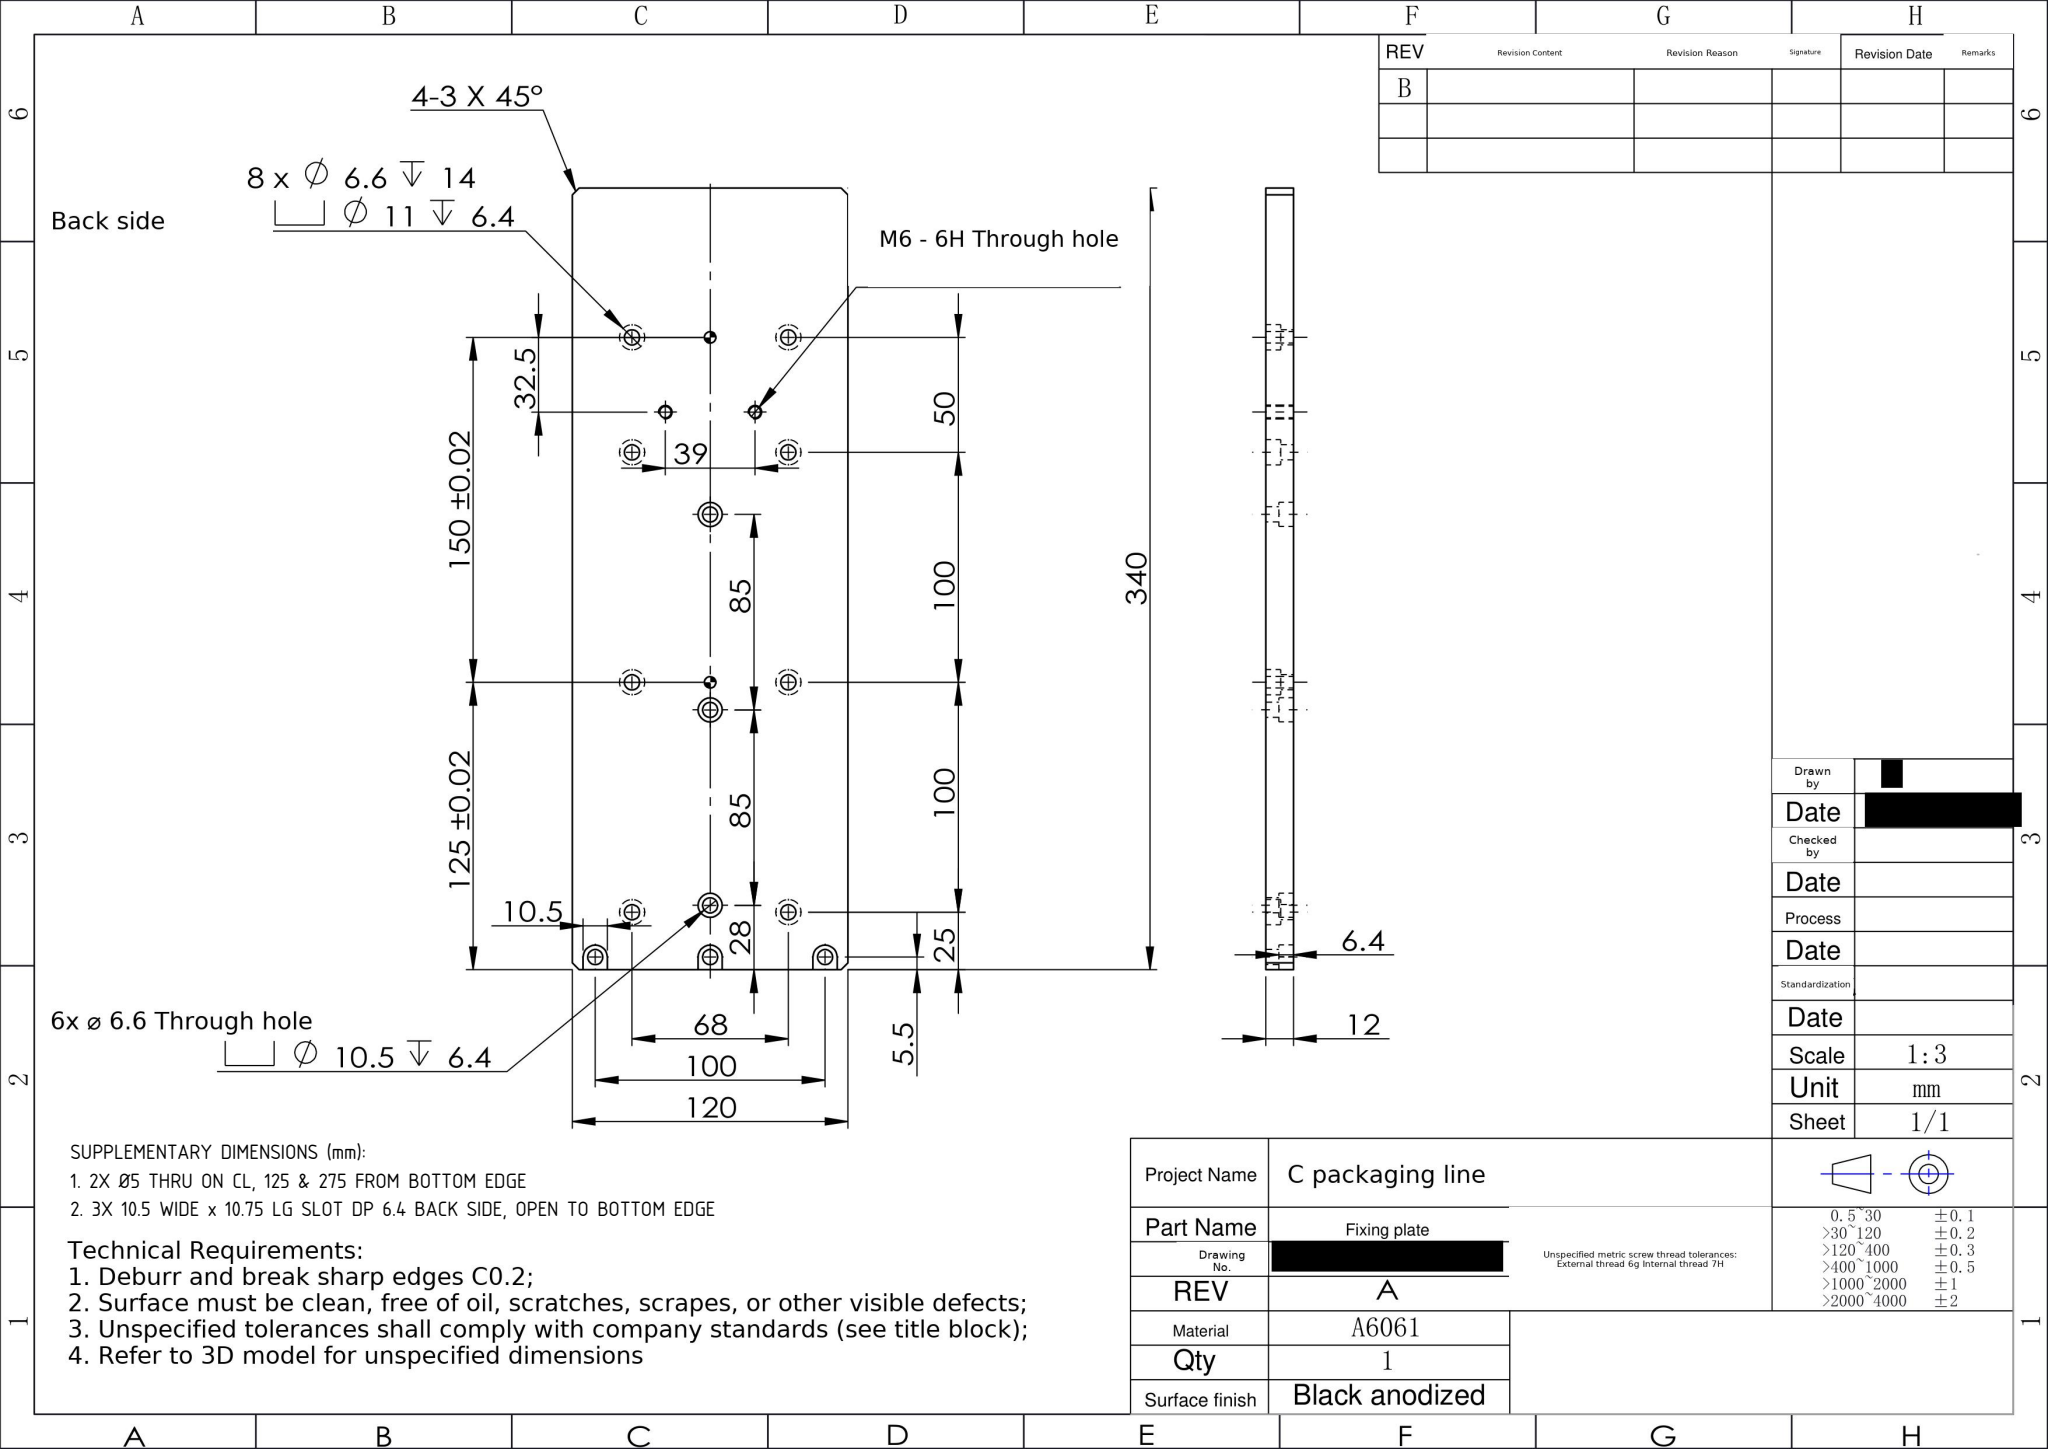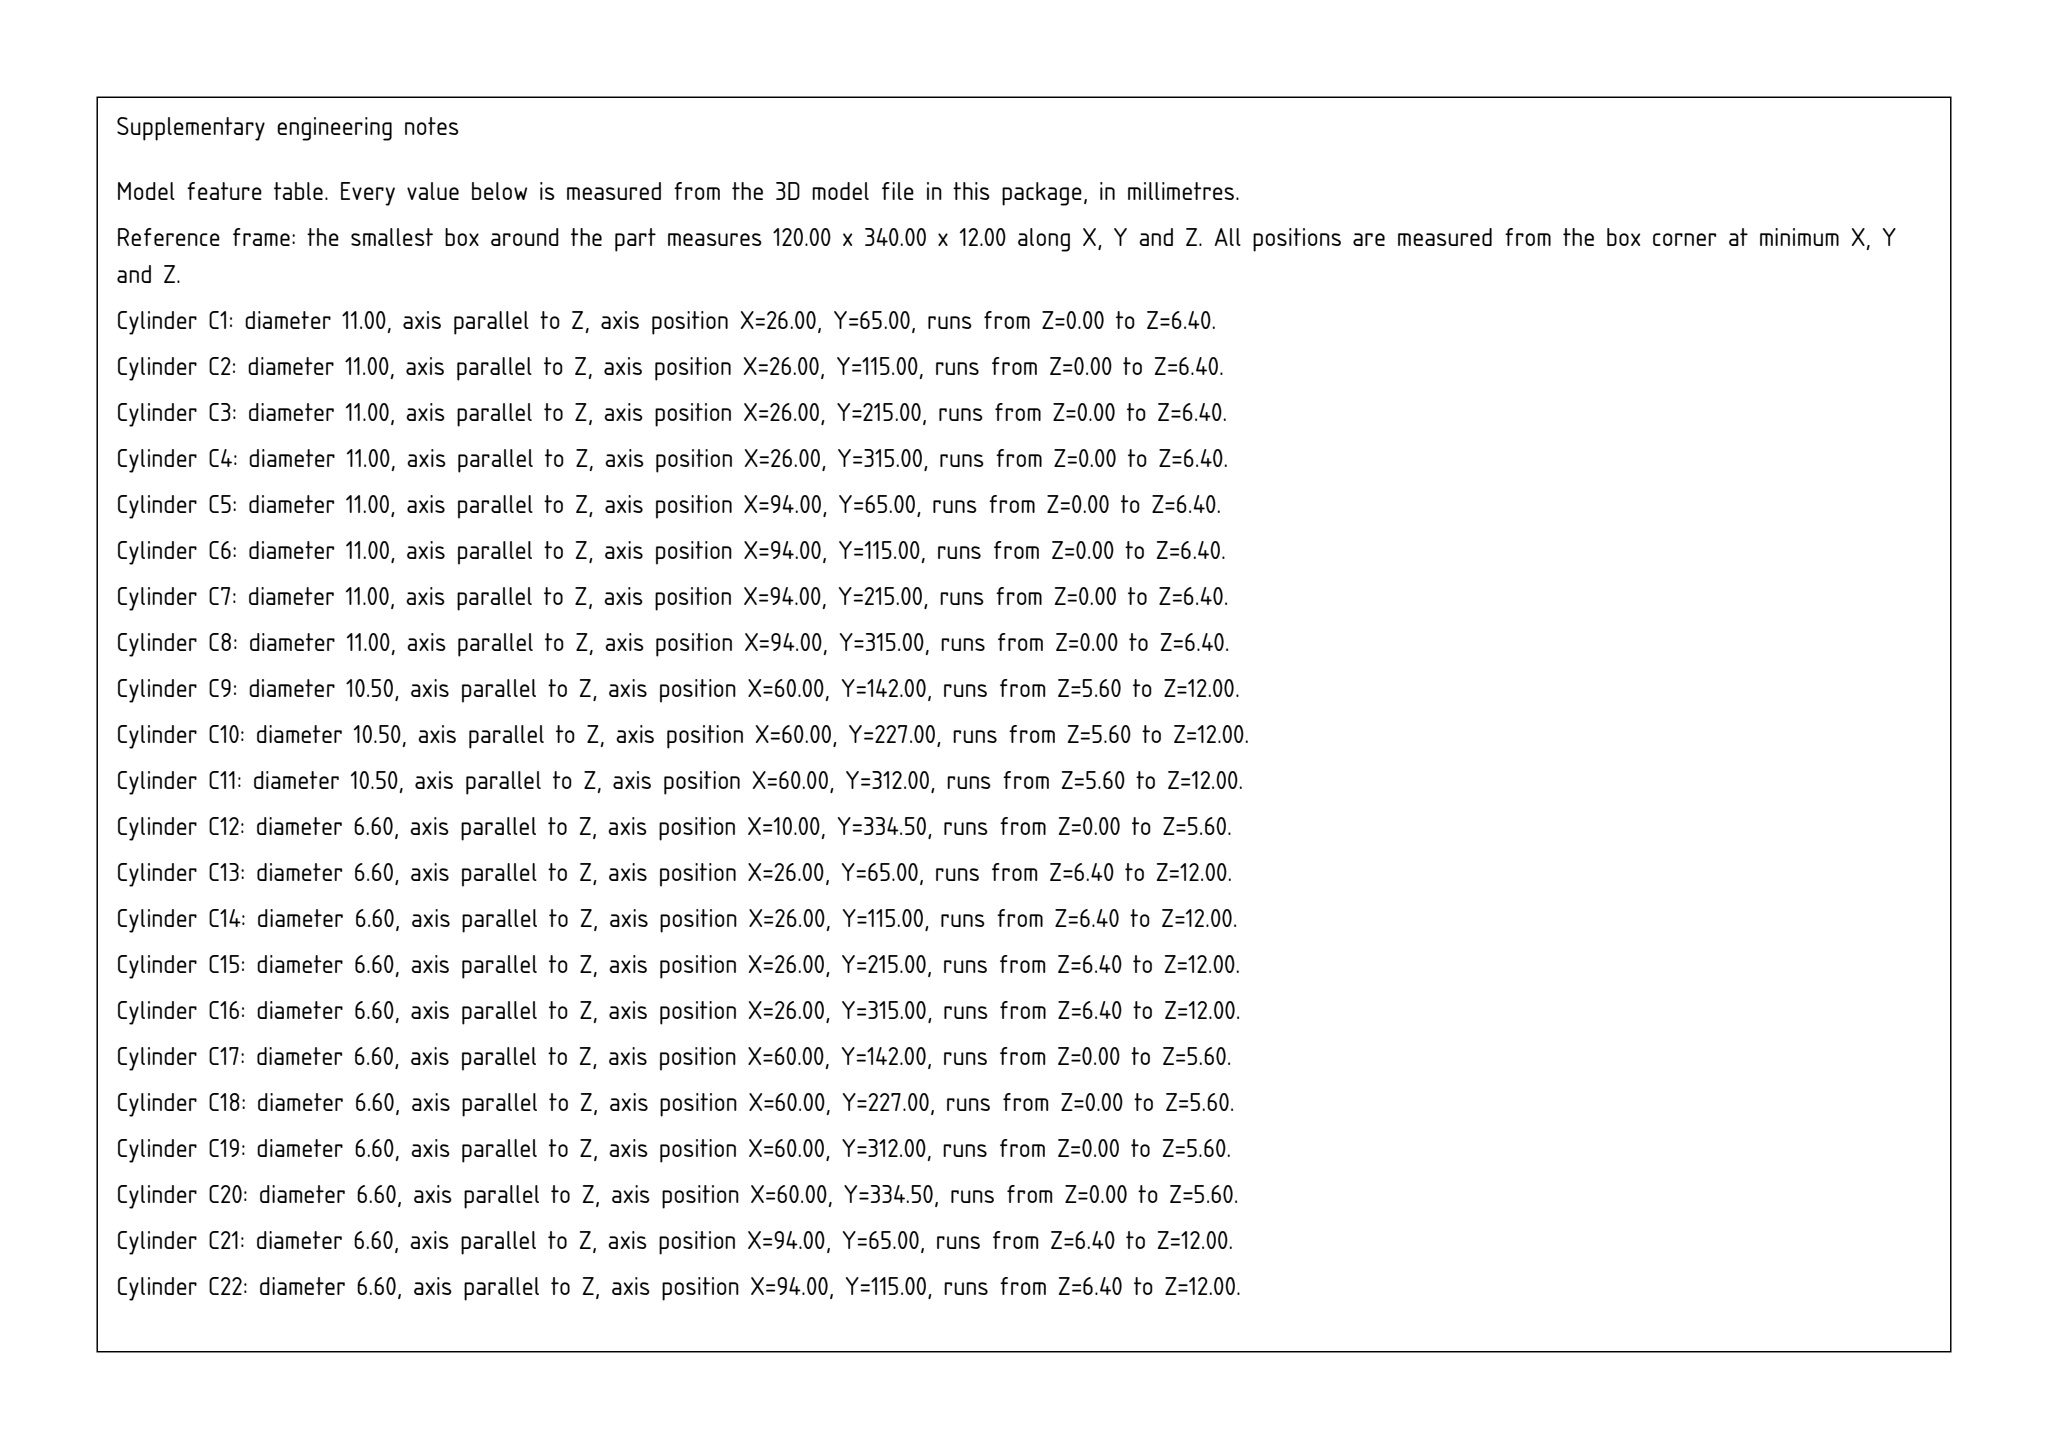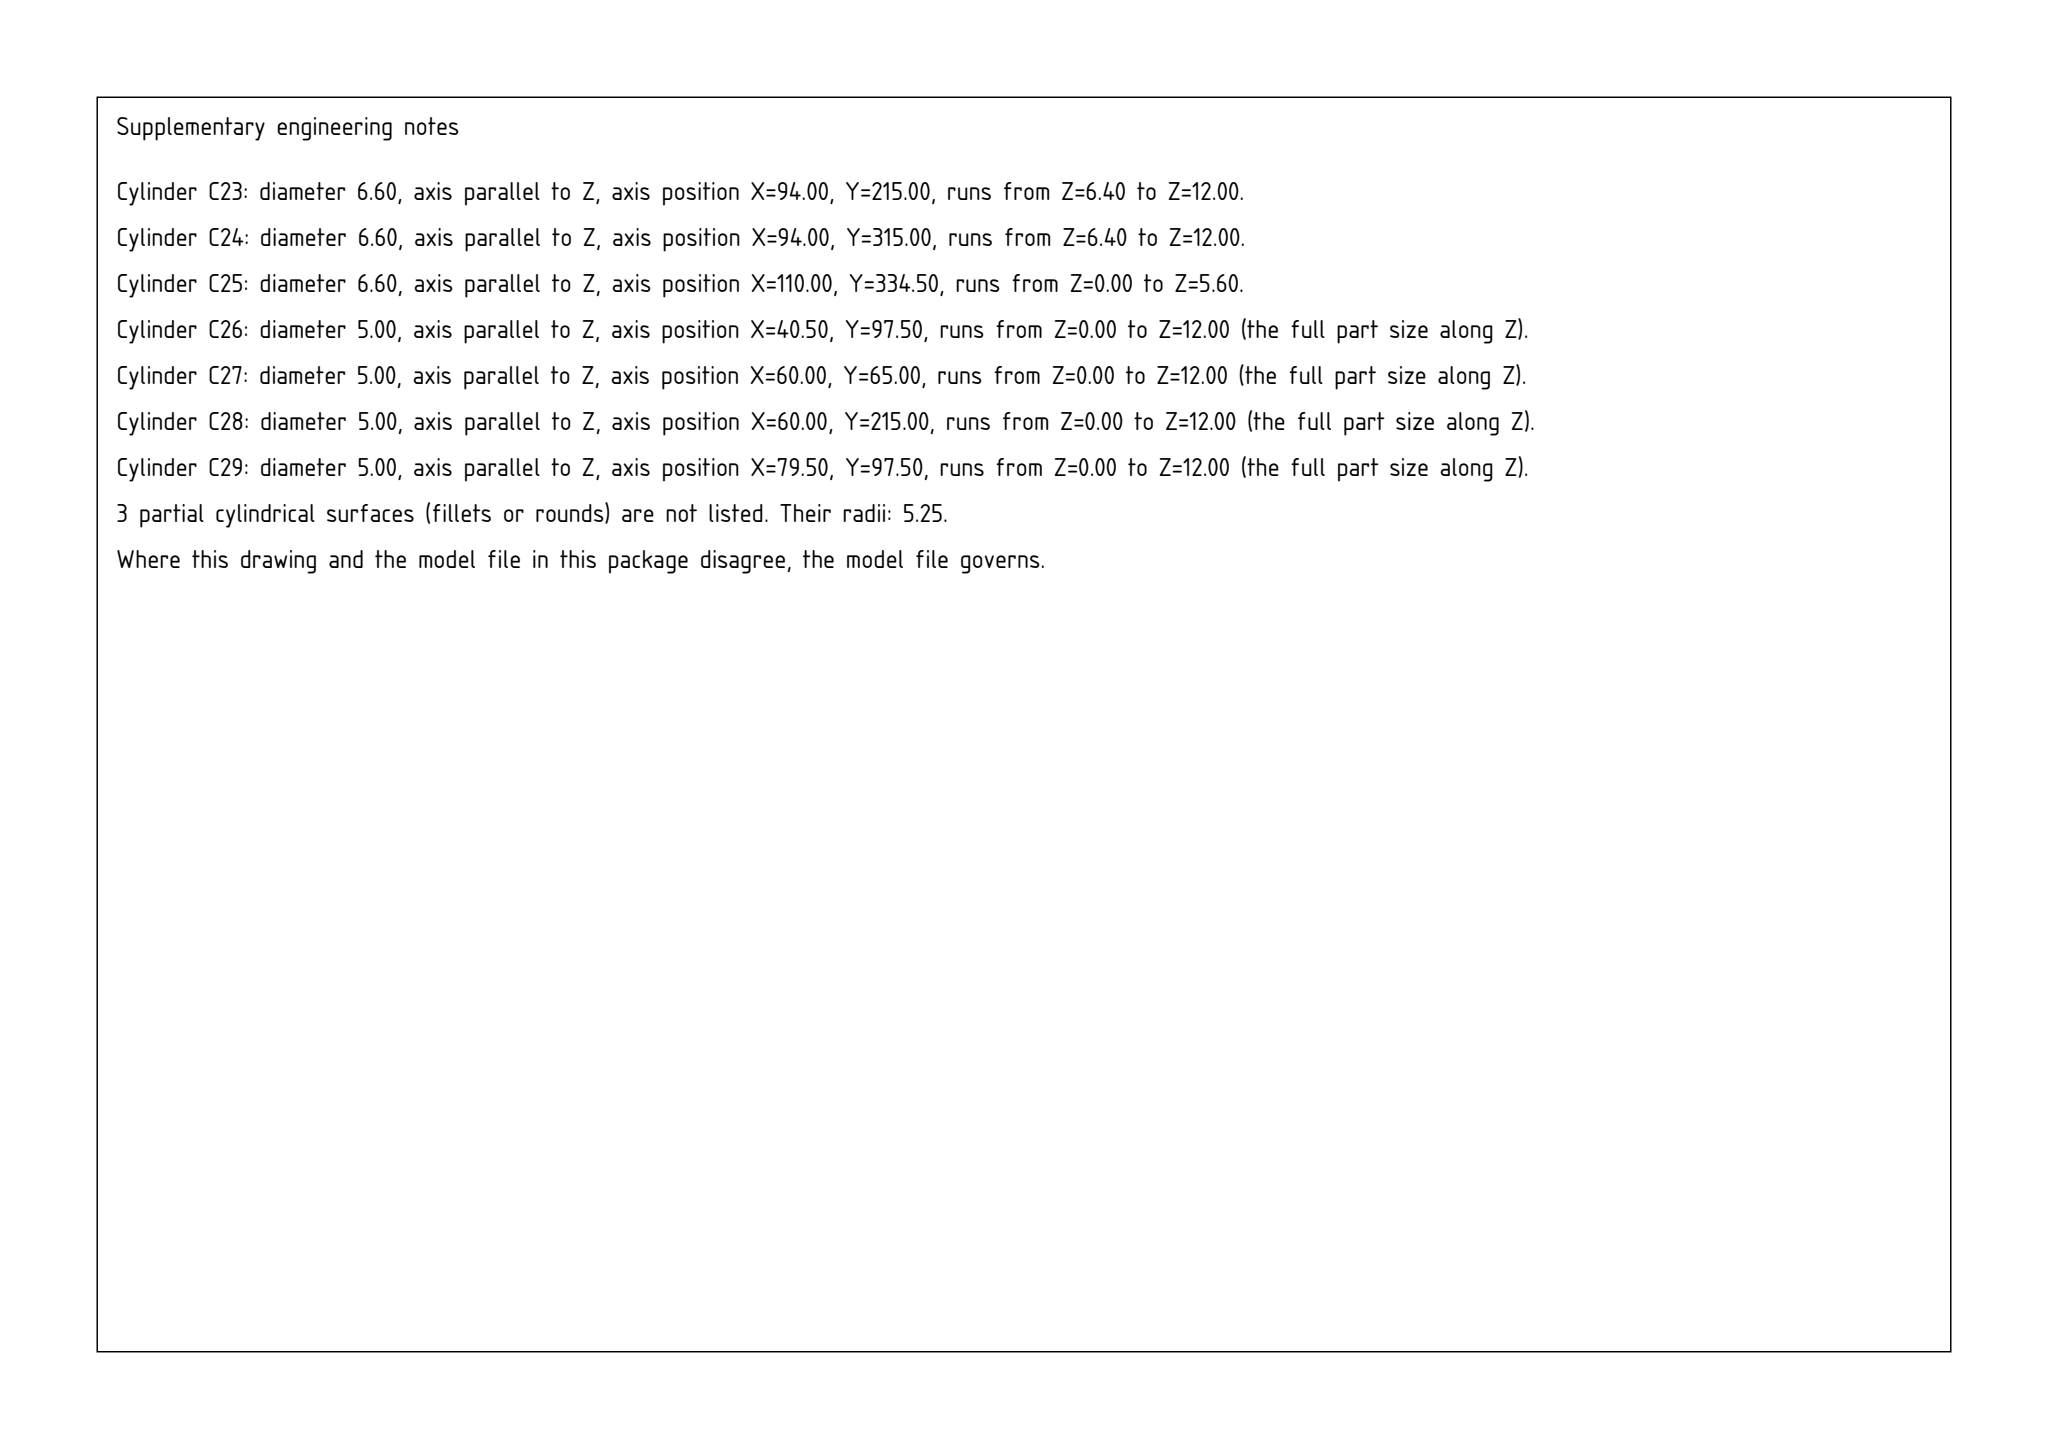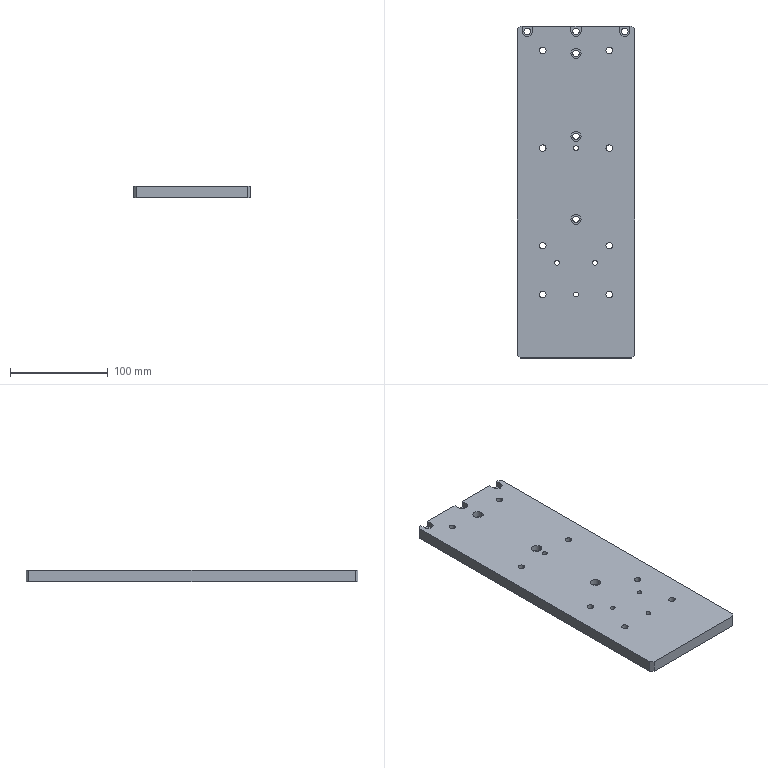Part | SolidWorks | mm | 1 solid | 91 faces | box 120 x 340 x 12 mm | volume 477291 mm3 | cylinder 61 | plane 30 | commonest cylinder face diameters 6.6 x28 11 x16 10.5 x9 5 x8
build123d program:
from build123d import *

# Parameters (mm, degrees)
SKETCH1_W                                       = 120
SKETCH1_H                                       = 340
BOSS_EXTRUDE1_DEPTH                             = 12
SKETCH6_W                                       = 270
SKETCH6_H                                       = 60
BOSS_EXTRUDE2_DEPTH                             = 12
M6_HEX_SOCKET_HEAD_CAP_SCREW_CBORE1_D           = 6.6
M6_HEX_SOCKET_HEAD_CAP_SCREW_CBORE1_DEPTH       = 14
M6_HEX_SOCKET_HEAD_CAP_SCREW_CBORE1_CBORE_D     = 11
M6_HEX_SOCKET_HEAD_CAP_SCREW_CBORE1_CBORE_DEPTH = 6.4
M6_HEX_SOCKET_HEAD_CAP_SCREW_CBORE1_TIP         = 1.983
F_5_0MM_DOWEL_PIN_HOLE1_D                       = 5
F_5_0MM_DOWEL_PIN_HOLE1_DEPTH                   = 14
F_5_0MM_DOWEL_PIN_HOLE1_TIP                     = 1.502
FILLET1_R                                       = 20
M5_TAPPED_HOLE1_D                               = 4.2
CHAMFER1_SIZE                                   = 3
M6_TAPPED_HOLE2_D                               = 5
SKETCH18_W                                      = 104.555
SKETCH18_H                                      = 178.513
SKETCH18_W_2                                    = 113.605
SKETCH18_H_2                                    = 153.389
CUT_EXTRUDE1_DEPTH                              = 218.414
M6_HEX_SOCKET_HEAD_CAP_SCREW_CBORE2_D           = 6.6
M6_HEX_SOCKET_HEAD_CAP_SCREW_CBORE2_CBORE_D     = 10.5
M6_HEX_SOCKET_HEAD_CAP_SCREW_CBORE2_CBORE_DEPTH = 6.4
SKETCH21_W                                      = 10.5
SKETCH21_H                                      = 16.339
CUT_EXTRUDE2_DEPTH                              = 6.4
LPATTERN1_COUNT                                 = 3
LPATTERN1_PITCH                                 = 50


with BuildPart() as part:
    # Sketch1 → Boss-Extrude1 (new body)
    with BuildSketch(Plane.XY):
        Rectangle(SKETCH1_W, SKETCH1_H)
    extrude(amount=BOSS_EXTRUDE1_DEPTH)

    # Sketch6 → Boss-Extrude2 (add)
    with BuildSketch(Plane(origin=(0, 0, 0), x_dir=(-1, 0, 0), z_dir=(0, 0, -1))):
        with Locations((0, -110)):
            Rectangle(SKETCH6_W, SKETCH6_H)
    extrude(amount=-BOSS_EXTRUDE2_DEPTH)

    # M6 Hex Socket Head Cap Screw CBORE1
    with Locations(Plane(origin=(0, 0, 0), x_dir=(-1, 0, 0), z_dir=(0, 0, -1))):
        with Locations((34, -105), (-34, -105), (34, -55), (-34, -55), (34, 45), (-34, 45), (34, 145), (-34, 145)):
            CounterBoreHole(M6_HEX_SOCKET_HEAD_CAP_SCREW_CBORE1_D / 2, M6_HEX_SOCKET_HEAD_CAP_SCREW_CBORE1_CBORE_D / 2, M6_HEX_SOCKET_HEAD_CAP_SCREW_CBORE1_CBORE_DEPTH, depth=M6_HEX_SOCKET_HEAD_CAP_SCREW_CBORE1_DEPTH)
            with Locations((0, 0, -(M6_HEX_SOCKET_HEAD_CAP_SCREW_CBORE1_DEPTH + M6_HEX_SOCKET_HEAD_CAP_SCREW_CBORE1_TIP / 2))):  # 118° drill point
                Cone(0, M6_HEX_SOCKET_HEAD_CAP_SCREW_CBORE1_D / 2, M6_HEX_SOCKET_HEAD_CAP_SCREW_CBORE1_TIP, mode=Mode.SUBTRACT)

    # 5.0mm Dowel Pin Hole1
    with Locations(Plane.XY.offset(12)):
        with Locations((0, 45), (0, -105)):
            Hole(F_5_0MM_DOWEL_PIN_HOLE1_D / 2, depth=F_5_0MM_DOWEL_PIN_HOLE1_DEPTH)
            with Locations((0, 0, -(F_5_0MM_DOWEL_PIN_HOLE1_DEPTH + F_5_0MM_DOWEL_PIN_HOLE1_TIP / 2))):  # 118° drill point
                Cone(0, F_5_0MM_DOWEL_PIN_HOLE1_D / 2, F_5_0MM_DOWEL_PIN_HOLE1_TIP, mode=Mode.SUBTRACT)

    # Fillet1
    fillet1_edges = [part.edges().sort_by_distance(p)[0] for p in [
        (60, -140, 6),
        (-60, -140, 6),
        (60, -80, 6),
        (-60, -80, 6),
    ]]
    fillet(fillet1_edges, radius=FILLET1_R)

    # M5 Tapped Hole1 (through all)
    with Locations(Plane(origin=(0, 0, 0), x_dir=(-1, 0, 0), z_dir=(0, 0, -1))):
        with Locations((91, -132), (91, -112), (116, -112), (116, -132), (104, -132), (129, -132), (129, -112), (104, -112)):
            m5_tapped_hole1 = Hole(M5_TAPPED_HOLE1_D / 2)

    # Mirror3: M5 Tapped Hole1 across plane
    add(m5_tapped_hole1.mirror(Plane.ZY), mode=Mode.SUBTRACT)

    # Chamfer1
    chamfer1_edges = [part.edges().sort_by_distance(p)[0] for p in [
        (-135, -140, 6),
        (135, -80, 6),
        (-135, -80, 6),
        (135, -140, 6),
        (60, -170, 6),
        (-60, -170, 6),
        (-60, 170, 6),
        (60, 170, 6),
    ]]
    chamfer(chamfer1_edges, length=CHAMFER1_SIZE)

    # M6 Tapped Hole2 (through all)
    with Locations(Plane(origin=(0, 0, 0), x_dir=(-1, 0, 0), z_dir=(0, 0, -1))):
        with Locations((-19.5, -72.5), (19.5, -72.5)):
            Hole(M6_TAPPED_HOLE2_D / 2)

    # Sketch18 → Cut-Extrude1 (cut, through all)
    with BuildSketch(Plane(origin=(0, 0, 0), x_dir=(-1, 0, 0), z_dir=(0, 0, -1))):
        with Locations((-112.278, -77.743)):
            Rectangle(SKETCH18_W, SKETCH18_H)
        with Locations((116.802, -90.305)):
            Rectangle(SKETCH18_W_2, SKETCH18_H_2)
    extrude(amount=-CUT_EXTRUDE1_DEPTH, mode=Mode.SUBTRACT)

    # M6 Hex Socket Head Cap Screw CBORE2 (through all)
    with Locations(Plane.XY.offset(12)):
        with Locations((-50, 164.5), (0, 142), (0, 164.5), (50, 164.5), (0, 57), (0, -28)):
            CounterBoreHole(M6_HEX_SOCKET_HEAD_CAP_SCREW_CBORE2_D / 2, M6_HEX_SOCKET_HEAD_CAP_SCREW_CBORE2_CBORE_D / 2, M6_HEX_SOCKET_HEAD_CAP_SCREW_CBORE2_CBORE_DEPTH)

    # Sketch21 → Cut-Extrude2 (cut)
    with BuildSketch(Plane.XY.offset(12)):
        with Locations((50, 172.669)):
            Rectangle(SKETCH21_W, SKETCH21_H)
    cut_extrude2 = extrude(amount=-CUT_EXTRUDE2_DEPTH, mode=Mode.SUBTRACT)

    # LPattern1: Cut-Extrude2 ×3
    with Locations(*[(-i * LPATTERN1_PITCH, 0, 0) for i in range(1, LPATTERN1_COUNT)]):
        add(cut_extrude2, mode=Mode.SUBTRACT)


solid = part.part